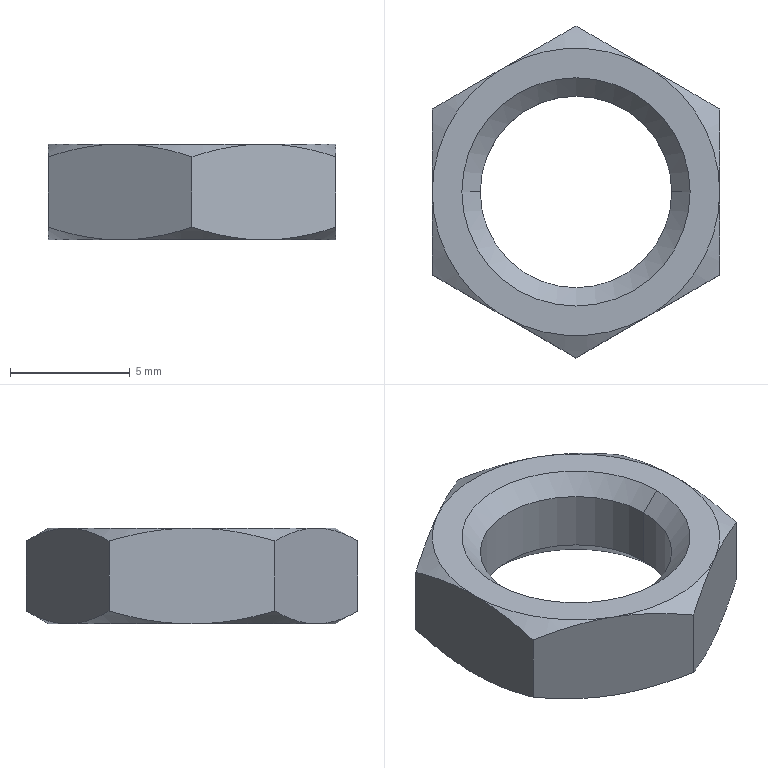Component | SolidWorks | RB0806-1_RB0806-3-1 | 1 solid | 26 faces | box 12 x 13.86 x 4 mm | volume 278 mm3 | cone 16 | plane 8 | cylinder 2 | commonest cylinder face diameters 8 x2
STEP:
#1=COLOUR_RGB('',0.7922,0.8196,0.9333);
#2=FILL_AREA_STYLE_COLOUR('',#1);
#3=FILL_AREA_STYLE('',(#2));
#4=SURFACE_STYLE_FILL_AREA(#3);
#5=SURFACE_SIDE_STYLE('',(#4));
#6=SURFACE_STYLE_USAGE(.BOTH.,#5);
#7=PRESENTATION_STYLE_ASSIGNMENT((#6));
#8=CARTESIAN_POINT('',(-0.6831,1.668,-1.143));
#9=VERTEX_POINT('',#8);
#10=CARTESIAN_POINT('',(-0.9981,1.668,-1.143));
#11=VERTEX_POINT('',#10);
#12=CARTESIAN_POINT('',(-0.8406,1.668,-1.143));
#13=DIRECTION('',(-0.,0.,1.));
#14=DIRECTION('',(-1.,0.,0.));
#15=AXIS2_PLACEMENT_3D('',#12,#13,#14);
#16=CIRCLE('',#15,0.1575);
#17=EDGE_CURVE('',#9,#11,#16,.T.);
#18=ORIENTED_EDGE('',*,*,#17,.F.);
#19=CARTESIAN_POINT('',(-0.653,1.668,-1.113));
#20=VERTEX_POINT('',#19);
#21=CARTESIAN_POINT('',(-0.668,1.668,-1.128));
#22=DIRECTION('',(0.7071,-0.,0.7071));
#23=VECTOR('',#22,39.37);
#24=LINE('',#21,#23);
#25=EDGE_CURVE('',#9,#20,#24,.T.);
#26=ORIENTED_EDGE('',*,*,#25,.T.);
#27=CARTESIAN_POINT('',(-1.028,1.668,-1.113));
#28=VERTEX_POINT('',#27);
#29=CARTESIAN_POINT('',(-0.8406,1.668,-1.113));
#30=DIRECTION('',(0.,-0.,-1.));
#31=DIRECTION('',(-1.,0.,0.));
#32=AXIS2_PLACEMENT_3D('',#29,#30,#31);
#33=CIRCLE('',#32,0.1876);
#34=EDGE_CURVE('',#28,#20,#33,.T.);
#35=ORIENTED_EDGE('',*,*,#34,.F.);
#36=CARTESIAN_POINT('',(-1.013,1.668,-1.128));
#37=DIRECTION('',(-0.7071,0.,0.7071));
#38=VECTOR('',#37,39.37);
#39=LINE('',#36,#38);
#40=EDGE_CURVE('',#11,#28,#39,.T.);
#41=ORIENTED_EDGE('',*,*,#40,.F.);
#42=EDGE_LOOP('',(#18,#26,#35,#41));
#43=FACE_OUTER_BOUND('',#42,.T.);
#44=CARTESIAN_POINT('',(-0.8406,1.668,-1.128));
#45=DIRECTION('',(-0.,0.,1.));
#46=DIRECTION('',(-1.,0.,0.));
#47=AXIS2_PLACEMENT_3D('',#44,#45,#46);
#48=CONICAL_SURFACE('',#47,0.1726,0.7854);
#49=ADVANCED_FACE('',(#43),#48,.F.);
#50=CARTESIAN_POINT('',(-0.6831,1.668,-1.24));
#51=VERTEX_POINT('',#50);
#52=CARTESIAN_POINT('',(-0.9981,1.668,-1.24));
#53=VERTEX_POINT('',#52);
#54=CARTESIAN_POINT('',(-0.8406,1.668,-1.24));
#55=DIRECTION('',(-0.,0.,1.));
#56=DIRECTION('',(1.,0.,0.));
#57=AXIS2_PLACEMENT_3D('',#54,#55,#56);
#58=CIRCLE('',#57,0.1575);
#59=EDGE_CURVE('',#51,#53,#58,.T.);
#60=ORIENTED_EDGE('',*,*,#59,.F.);
#61=CARTESIAN_POINT('',(-0.6831,1.668,-1.192));
#62=DIRECTION('',(-0.,0.,1.));
#63=VECTOR('',#62,39.37);
#64=LINE('',#61,#63);
#65=EDGE_CURVE('',#51,#9,#64,.T.);
#66=ORIENTED_EDGE('',*,*,#65,.T.);
#67=ORIENTED_EDGE('',*,*,#17,.T.);
#68=CARTESIAN_POINT('',(-0.9981,1.668,-1.192));
#69=DIRECTION('',(-0.,0.,1.));
#70=VECTOR('',#69,39.37);
#71=LINE('',#68,#70);
#72=EDGE_CURVE('',#53,#11,#71,.T.);
#73=ORIENTED_EDGE('',*,*,#72,.F.);
#74=EDGE_LOOP('',(#60,#66,#67,#73));
#75=FACE_OUTER_BOUND('',#74,.T.);
#76=CARTESIAN_POINT('',(-0.8406,1.668,-1.192));
#77=DIRECTION('',(-0.,0.,1.));
#78=DIRECTION('',(-1.,0.,0.));
#79=AXIS2_PLACEMENT_3D('',#76,#77,#78);
#80=CYLINDRICAL_SURFACE('',#79,0.1575);
#81=ADVANCED_FACE('',(#75),#80,.F.);
#82=ORIENTED_EDGE('',*,*,#59,.T.);
#83=CARTESIAN_POINT('',(-1.028,1.668,-1.27));
#84=VERTEX_POINT('',#83);
#85=CARTESIAN_POINT('',(-1.013,1.668,-1.255));
#86=DIRECTION('',(-0.7071,-0.,-0.7071));
#87=VECTOR('',#86,39.37);
#88=LINE('',#85,#87);
#89=EDGE_CURVE('',#53,#84,#88,.T.);
#90=ORIENTED_EDGE('',*,*,#89,.T.);
#91=CARTESIAN_POINT('',(-0.653,1.668,-1.27));
#92=VERTEX_POINT('',#91);
#93=CARTESIAN_POINT('',(-0.8406,1.668,-1.27));
#94=DIRECTION('',(-0.,0.,1.));
#95=DIRECTION('',(1.,0.,0.));
#96=AXIS2_PLACEMENT_3D('',#93,#94,#95);
#97=CIRCLE('',#96,0.1876);
#98=EDGE_CURVE('',#92,#84,#97,.T.);
#99=ORIENTED_EDGE('',*,*,#98,.F.);
#100=CARTESIAN_POINT('',(-0.668,1.668,-1.255));
#101=DIRECTION('',(0.7071,-0.,-0.7071));
#102=VECTOR('',#101,39.37);
#103=LINE('',#100,#102);
#104=EDGE_CURVE('',#51,#92,#103,.T.);
#105=ORIENTED_EDGE('',*,*,#104,.F.);
#106=EDGE_LOOP('',(#82,#90,#99,#105));
#107=FACE_OUTER_BOUND('',#106,.T.);
#108=CARTESIAN_POINT('',(-0.8406,1.668,-1.255));
#109=DIRECTION('',(0.,-0.,-1.));
#110=DIRECTION('',(1.,0.,0.));
#111=AXIS2_PLACEMENT_3D('',#108,#109,#110);
#112=CONICAL_SURFACE('',#111,0.1726,0.7854);
#113=ADVANCED_FACE('',(#107),#112,.F.);
#114=ORIENTED_EDGE('',*,*,#34,.T.);
#115=CARTESIAN_POINT('',(-0.8406,1.668,-1.113));
#116=DIRECTION('',(0.,-0.,-1.));
#117=DIRECTION('',(-1.,0.,0.));
#118=AXIS2_PLACEMENT_3D('',#115,#116,#117);
#119=CIRCLE('',#118,0.1876);
#120=EDGE_CURVE('',#20,#28,#119,.T.);
#121=ORIENTED_EDGE('',*,*,#120,.T.);
#122=EDGE_LOOP('',(#114,#121));
#123=FACE_BOUND('',#122,.T.);
#124=CARTESIAN_POINT('',(-0.6044,1.668,-1.113));
#125=VERTEX_POINT('',#124);
#126=CARTESIAN_POINT('',(-0.7225,1.872,-1.113));
#127=VERTEX_POINT('',#126);
#128=CARTESIAN_POINT('',(-0.8406,1.668,-1.113));
#129=DIRECTION('',(-0.,0.,1.));
#130=DIRECTION('',(1.,0.,0.));
#131=AXIS2_PLACEMENT_3D('',#128,#129,#130);
#132=CIRCLE('',#131,0.2362);
#133=EDGE_CURVE('',#125,#127,#132,.T.);
#134=ORIENTED_EDGE('',*,*,#133,.T.);
#135=CARTESIAN_POINT('',(-0.9587,1.872,-1.113));
#136=VERTEX_POINT('',#135);
#137=CARTESIAN_POINT('',(-0.8406,1.668,-1.113));
#138=DIRECTION('',(-0.,0.,1.));
#139=DIRECTION('',(1.,0.,0.));
#140=AXIS2_PLACEMENT_3D('',#137,#138,#139);
#141=CIRCLE('',#140,0.2362);
#142=EDGE_CURVE('',#127,#136,#141,.T.);
#143=ORIENTED_EDGE('',*,*,#142,.T.);
#144=CARTESIAN_POINT('',(-1.077,1.668,-1.113));
#145=VERTEX_POINT('',#144);
#146=CARTESIAN_POINT('',(-0.8406,1.668,-1.113));
#147=DIRECTION('',(-0.,0.,1.));
#148=DIRECTION('',(1.,0.,0.));
#149=AXIS2_PLACEMENT_3D('',#146,#147,#148);
#150=CIRCLE('',#149,0.2362);
#151=EDGE_CURVE('',#136,#145,#150,.T.);
#152=ORIENTED_EDGE('',*,*,#151,.T.);
#153=CARTESIAN_POINT('',(-0.9587,1.463,-1.113));
#154=VERTEX_POINT('',#153);
#155=CARTESIAN_POINT('',(-0.8406,1.668,-1.113));
#156=DIRECTION('',(-0.,0.,1.));
#157=DIRECTION('',(1.,0.,0.));
#158=AXIS2_PLACEMENT_3D('',#155,#156,#157);
#159=CIRCLE('',#158,0.2362);
#160=EDGE_CURVE('',#145,#154,#159,.T.);
#161=ORIENTED_EDGE('',*,*,#160,.T.);
#162=CARTESIAN_POINT('',(-0.7225,1.463,-1.113));
#163=VERTEX_POINT('',#162);
#164=CARTESIAN_POINT('',(-0.8406,1.668,-1.113));
#165=DIRECTION('',(-0.,0.,1.));
#166=DIRECTION('',(1.,-0.,0.));
#167=AXIS2_PLACEMENT_3D('',#164,#165,#166);
#168=CIRCLE('',#167,0.2362);
#169=EDGE_CURVE('',#154,#163,#168,.T.);
#170=ORIENTED_EDGE('',*,*,#169,.T.);
#171=CARTESIAN_POINT('',(-0.8406,1.668,-1.113));
#172=DIRECTION('',(-0.,0.,1.));
#173=DIRECTION('',(1.,-0.,0.));
#174=AXIS2_PLACEMENT_3D('',#171,#172,#173);
#175=CIRCLE('',#174,0.2362);
#176=EDGE_CURVE('',#163,#125,#175,.T.);
#177=ORIENTED_EDGE('',*,*,#176,.T.);
#178=EDGE_LOOP('',(#134,#143,#152,#161,#170,#177));
#179=FACE_OUTER_BOUND('',#178,.T.);
#180=CARTESIAN_POINT('',(-0.8406,1.865,-1.113));
#181=DIRECTION('',(-0.,0.,1.));
#182=DIRECTION('',(-1.,0.,-0.));
#183=AXIS2_PLACEMENT_3D('',#180,#181,#182);
#184=PLANE('',#183);
#185=ADVANCED_FACE('',(#123,#179),#184,.T.);
#186=ORIENTED_EDGE('',*,*,#25,.F.);
#187=CARTESIAN_POINT('',(-0.8406,1.668,-1.143));
#188=DIRECTION('',(-0.,0.,1.));
#189=DIRECTION('',(-1.,0.,0.));
#190=AXIS2_PLACEMENT_3D('',#187,#188,#189);
#191=CIRCLE('',#190,0.1575);
#192=EDGE_CURVE('',#11,#9,#191,.T.);
#193=ORIENTED_EDGE('',*,*,#192,.F.);
#194=ORIENTED_EDGE('',*,*,#40,.T.);
#195=ORIENTED_EDGE('',*,*,#120,.F.);
#196=EDGE_LOOP('',(#186,#193,#194,#195));
#197=FACE_OUTER_BOUND('',#196,.T.);
#198=CARTESIAN_POINT('',(-0.8406,1.668,-1.128));
#199=DIRECTION('',(-0.,0.,1.));
#200=DIRECTION('',(-1.,0.,0.));
#201=AXIS2_PLACEMENT_3D('',#198,#199,#200);
#202=CONICAL_SURFACE('',#201,0.1726,0.7854);
#203=ADVANCED_FACE('',(#197),#202,.F.);
#204=ORIENTED_EDGE('',*,*,#142,.F.);
#205=CARTESIAN_POINT('',(-0.8406,1.941,-1.134));
#206=VERTEX_POINT('',#205);
#207=CARTESIAN_POINT('',(-0.7225,1.872,-1.113));
#208=CARTESIAN_POINT('',(-0.7628,1.896,-1.113));
#209=CARTESIAN_POINT('',(-0.802,1.918,-1.121));
#210=CARTESIAN_POINT('',(-0.8406,1.941,-1.134));
#211=B_SPLINE_CURVE_WITH_KNOTS('',3,(#207,#208,#209,#210),.UNSPECIFIED.,.F.,.F.,(4,4),(0.,0.003505),.UNSPECIFIED.);
#212=EDGE_CURVE('',#127,#206,#211,.T.);
#213=ORIENTED_EDGE('',*,*,#212,.T.);
#214=CARTESIAN_POINT('',(-0.8406,1.941,-1.134));
#215=CARTESIAN_POINT('',(-0.8792,1.918,-1.121));
#216=CARTESIAN_POINT('',(-0.9184,1.896,-1.113));
#217=CARTESIAN_POINT('',(-0.9587,1.872,-1.113));
#218=B_SPLINE_CURVE_WITH_KNOTS('',3,(#214,#215,#216,#217),.UNSPECIFIED.,.F.,.F.,(4,4),(0.,0.003505),.UNSPECIFIED.);
#219=EDGE_CURVE('',#206,#136,#218,.T.);
#220=ORIENTED_EDGE('',*,*,#219,.T.);
#221=EDGE_LOOP('',(#204,#213,#220));
#222=FACE_OUTER_BOUND('',#221,.T.);
#223=CARTESIAN_POINT('',(-0.8406,1.668,-1.134));
#224=DIRECTION('',(0.,-0.,-1.));
#225=DIRECTION('',(1.,0.,0.));
#226=AXIS2_PLACEMENT_3D('',#223,#224,#225);
#227=CONICAL_SURFACE('',#226,0.273,1.047);
#228=ADVANCED_FACE('',(#222),#227,.T.);
#229=CARTESIAN_POINT('',(-0.6044,1.804,-1.134));
#230=VERTEX_POINT('',#229);
#231=CARTESIAN_POINT('',(-0.6044,1.804,-1.134));
#232=CARTESIAN_POINT('',(-0.6429,1.827,-1.121));
#233=CARTESIAN_POINT('',(-0.6822,1.849,-1.113));
#234=CARTESIAN_POINT('',(-0.7225,1.872,-1.113));
#235=B_SPLINE_CURVE_WITH_KNOTS('',3,(#231,#232,#233,#234),.UNSPECIFIED.,.F.,.F.,(4,4),(0.,0.003505),.UNSPECIFIED.);
#236=EDGE_CURVE('',#230,#127,#235,.T.);
#237=ORIENTED_EDGE('',*,*,#236,.T.);
#238=ORIENTED_EDGE('',*,*,#133,.F.);
#239=CARTESIAN_POINT('',(-0.6044,1.668,-1.113));
#240=CARTESIAN_POINT('',(-0.6044,1.714,-1.113));
#241=CARTESIAN_POINT('',(-0.6044,1.76,-1.121));
#242=CARTESIAN_POINT('',(-0.6044,1.804,-1.134));
#243=B_SPLINE_CURVE_WITH_KNOTS('',3,(#239,#240,#241,#242),.UNSPECIFIED.,.F.,.F.,(4,4),(0.,0.003505),.UNSPECIFIED.);
#244=EDGE_CURVE('',#125,#230,#243,.T.);
#245=ORIENTED_EDGE('',*,*,#244,.T.);
#246=EDGE_LOOP('',(#237,#238,#245));
#247=FACE_OUTER_BOUND('',#246,.T.);
#248=CARTESIAN_POINT('',(-0.8406,1.668,-1.134));
#249=DIRECTION('',(0.,-0.,-1.));
#250=DIRECTION('',(1.,0.,0.));
#251=AXIS2_PLACEMENT_3D('',#248,#249,#250);
#252=CONICAL_SURFACE('',#251,0.273,1.047);
#253=ADVANCED_FACE('',(#247),#252,.T.);
#254=ORIENTED_EDGE('',*,*,#176,.F.);
#255=CARTESIAN_POINT('',(-0.6044,1.532,-1.134));
#256=VERTEX_POINT('',#255);
#257=CARTESIAN_POINT('',(-0.7225,1.463,-1.113));
#258=CARTESIAN_POINT('',(-0.6822,1.487,-1.113));
#259=CARTESIAN_POINT('',(-0.6429,1.509,-1.121));
#260=CARTESIAN_POINT('',(-0.6044,1.532,-1.134));
#261=B_SPLINE_CURVE_WITH_KNOTS('',3,(#257,#258,#259,#260),.UNSPECIFIED.,.F.,.F.,(4,4),(0.,0.003505),.UNSPECIFIED.);
#262=EDGE_CURVE('',#163,#256,#261,.T.);
#263=ORIENTED_EDGE('',*,*,#262,.T.);
#264=CARTESIAN_POINT('',(-0.6044,1.532,-1.134));
#265=CARTESIAN_POINT('',(-0.6044,1.576,-1.121));
#266=CARTESIAN_POINT('',(-0.6044,1.621,-1.113));
#267=CARTESIAN_POINT('',(-0.6044,1.668,-1.113));
#268=B_SPLINE_CURVE_WITH_KNOTS('',3,(#264,#265,#266,#267),.UNSPECIFIED.,.F.,.F.,(4,4),(0.,0.003505),.UNSPECIFIED.);
#269=EDGE_CURVE('',#256,#125,#268,.T.);
#270=ORIENTED_EDGE('',*,*,#269,.T.);
#271=EDGE_LOOP('',(#254,#263,#270));
#272=FACE_OUTER_BOUND('',#271,.T.);
#273=CARTESIAN_POINT('',(-0.8406,1.668,-1.134));
#274=DIRECTION('',(0.,-0.,-1.));
#275=DIRECTION('',(1.,0.,0.));
#276=AXIS2_PLACEMENT_3D('',#273,#274,#275);
#277=CONICAL_SURFACE('',#276,0.273,1.047);
#278=ADVANCED_FACE('',(#272),#277,.T.);
#279=CARTESIAN_POINT('',(-0.8406,1.395,-1.134));
#280=VERTEX_POINT('',#279);
#281=CARTESIAN_POINT('',(-0.8406,1.395,-1.134));
#282=CARTESIAN_POINT('',(-0.802,1.417,-1.121));
#283=CARTESIAN_POINT('',(-0.7628,1.44,-1.113));
#284=CARTESIAN_POINT('',(-0.7225,1.463,-1.113));
#285=B_SPLINE_CURVE_WITH_KNOTS('',3,(#281,#282,#283,#284),.UNSPECIFIED.,.F.,.F.,(4,4),(0.,0.003505),.UNSPECIFIED.);
#286=EDGE_CURVE('',#280,#163,#285,.T.);
#287=ORIENTED_EDGE('',*,*,#286,.T.);
#288=ORIENTED_EDGE('',*,*,#169,.F.);
#289=CARTESIAN_POINT('',(-0.9587,1.463,-1.113));
#290=CARTESIAN_POINT('',(-0.9184,1.44,-1.113));
#291=CARTESIAN_POINT('',(-0.8792,1.417,-1.121));
#292=CARTESIAN_POINT('',(-0.8406,1.395,-1.134));
#293=B_SPLINE_CURVE_WITH_KNOTS('',3,(#289,#290,#291,#292),.UNSPECIFIED.,.F.,.F.,(4,4),(0.,0.003505),.UNSPECIFIED.);
#294=EDGE_CURVE('',#154,#280,#293,.T.);
#295=ORIENTED_EDGE('',*,*,#294,.T.);
#296=EDGE_LOOP('',(#287,#288,#295));
#297=FACE_OUTER_BOUND('',#296,.T.);
#298=CARTESIAN_POINT('',(-0.8406,1.668,-1.134));
#299=DIRECTION('',(0.,-0.,-1.));
#300=DIRECTION('',(1.,0.,0.));
#301=AXIS2_PLACEMENT_3D('',#298,#299,#300);
#302=CONICAL_SURFACE('',#301,0.273,1.047);
#303=ADVANCED_FACE('',(#297),#302,.T.);
#304=ORIENTED_EDGE('',*,*,#160,.F.);
#305=CARTESIAN_POINT('',(-1.077,1.532,-1.134));
#306=VERTEX_POINT('',#305);
#307=CARTESIAN_POINT('',(-1.077,1.668,-1.113));
#308=CARTESIAN_POINT('',(-1.077,1.621,-1.113));
#309=CARTESIAN_POINT('',(-1.077,1.576,-1.121));
#310=CARTESIAN_POINT('',(-1.077,1.532,-1.134));
#311=B_SPLINE_CURVE_WITH_KNOTS('',3,(#307,#308,#309,#310),.UNSPECIFIED.,.F.,.F.,(4,4),(0.,0.003505),.UNSPECIFIED.);
#312=EDGE_CURVE('',#145,#306,#311,.T.);
#313=ORIENTED_EDGE('',*,*,#312,.T.);
#314=CARTESIAN_POINT('',(-1.077,1.532,-1.134));
#315=CARTESIAN_POINT('',(-1.038,1.509,-1.121));
#316=CARTESIAN_POINT('',(-0.999,1.487,-1.113));
#317=CARTESIAN_POINT('',(-0.9587,1.463,-1.113));
#318=B_SPLINE_CURVE_WITH_KNOTS('',3,(#314,#315,#316,#317),.UNSPECIFIED.,.F.,.F.,(4,4),(0.,0.003505),.UNSPECIFIED.);
#319=EDGE_CURVE('',#306,#154,#318,.T.);
#320=ORIENTED_EDGE('',*,*,#319,.T.);
#321=EDGE_LOOP('',(#304,#313,#320));
#322=FACE_OUTER_BOUND('',#321,.T.);
#323=CARTESIAN_POINT('',(-0.8406,1.668,-1.134));
#324=DIRECTION('',(0.,-0.,-1.));
#325=DIRECTION('',(1.,0.,0.));
#326=AXIS2_PLACEMENT_3D('',#323,#324,#325);
#327=CONICAL_SURFACE('',#326,0.273,1.047);
#328=ADVANCED_FACE('',(#322),#327,.T.);
#329=CARTESIAN_POINT('',(-1.077,1.804,-1.134));
#330=VERTEX_POINT('',#329);
#331=CARTESIAN_POINT('',(-1.077,1.804,-1.134));
#332=CARTESIAN_POINT('',(-1.077,1.76,-1.121));
#333=CARTESIAN_POINT('',(-1.077,1.714,-1.113));
#334=CARTESIAN_POINT('',(-1.077,1.668,-1.113));
#335=B_SPLINE_CURVE_WITH_KNOTS('',3,(#331,#332,#333,#334),.UNSPECIFIED.,.F.,.F.,(4,4),(0.,0.003505),.UNSPECIFIED.);
#336=EDGE_CURVE('',#330,#145,#335,.T.);
#337=ORIENTED_EDGE('',*,*,#336,.T.);
#338=ORIENTED_EDGE('',*,*,#151,.F.);
#339=CARTESIAN_POINT('',(-0.9587,1.872,-1.113));
#340=CARTESIAN_POINT('',(-0.999,1.849,-1.113));
#341=CARTESIAN_POINT('',(-1.038,1.827,-1.121));
#342=CARTESIAN_POINT('',(-1.077,1.804,-1.134));
#343=B_SPLINE_CURVE_WITH_KNOTS('',3,(#339,#340,#341,#342),.UNSPECIFIED.,.F.,.F.,(4,4),(0.,0.003505),.UNSPECIFIED.);
#344=EDGE_CURVE('',#136,#330,#343,.T.);
#345=ORIENTED_EDGE('',*,*,#344,.T.);
#346=EDGE_LOOP('',(#337,#338,#345));
#347=FACE_OUTER_BOUND('',#346,.T.);
#348=CARTESIAN_POINT('',(-0.8406,1.668,-1.134));
#349=DIRECTION('',(0.,-0.,-1.));
#350=DIRECTION('',(1.,0.,0.));
#351=AXIS2_PLACEMENT_3D('',#348,#349,#350);
#352=CONICAL_SURFACE('',#351,0.273,1.047);
#353=ADVANCED_FACE('',(#347),#352,.T.);
#354=ORIENTED_EDGE('',*,*,#65,.F.);
#355=CARTESIAN_POINT('',(-0.8406,1.668,-1.24));
#356=DIRECTION('',(-0.,0.,1.));
#357=DIRECTION('',(1.,0.,0.));
#358=AXIS2_PLACEMENT_3D('',#355,#356,#357);
#359=CIRCLE('',#358,0.1575);
#360=EDGE_CURVE('',#53,#51,#359,.T.);
#361=ORIENTED_EDGE('',*,*,#360,.F.);
#362=ORIENTED_EDGE('',*,*,#72,.T.);
#363=ORIENTED_EDGE('',*,*,#192,.T.);
#364=EDGE_LOOP('',(#354,#361,#362,#363));
#365=FACE_OUTER_BOUND('',#364,.T.);
#366=CARTESIAN_POINT('',(-0.8406,1.668,-1.192));
#367=DIRECTION('',(-0.,0.,1.));
#368=DIRECTION('',(-1.,0.,0.));
#369=AXIS2_PLACEMENT_3D('',#366,#367,#368);
#370=CYLINDRICAL_SURFACE('',#369,0.1575);
#371=ADVANCED_FACE('',(#365),#370,.F.);
#372=CARTESIAN_POINT('',(-0.6044,1.804,-1.249));
#373=VERTEX_POINT('',#372);
#374=CARTESIAN_POINT('',(-0.6044,1.804,-1.27));
#375=DIRECTION('',(-0.,0.,1.));
#376=VECTOR('',#375,39.37);
#377=LINE('',#374,#376);
#378=EDGE_CURVE('',#373,#230,#377,.T.);
#379=ORIENTED_EDGE('',*,*,#378,.F.);
#380=CARTESIAN_POINT('',(-0.7225,1.872,-1.27));
#381=VERTEX_POINT('',#380);
#382=CARTESIAN_POINT('',(-0.7225,1.872,-1.27));
#383=CARTESIAN_POINT('',(-0.6822,1.849,-1.27));
#384=CARTESIAN_POINT('',(-0.6429,1.827,-1.262));
#385=CARTESIAN_POINT('',(-0.6044,1.804,-1.249));
#386=B_SPLINE_CURVE_WITH_KNOTS('',3,(#382,#383,#384,#385),.UNSPECIFIED.,.F.,.F.,(4,4),(0.,0.003505),.UNSPECIFIED.);
#387=EDGE_CURVE('',#381,#373,#386,.T.);
#388=ORIENTED_EDGE('',*,*,#387,.F.);
#389=CARTESIAN_POINT('',(-0.8406,1.941,-1.249));
#390=VERTEX_POINT('',#389);
#391=CARTESIAN_POINT('',(-0.8406,1.941,-1.249));
#392=CARTESIAN_POINT('',(-0.802,1.918,-1.262));
#393=CARTESIAN_POINT('',(-0.7628,1.896,-1.27));
#394=CARTESIAN_POINT('',(-0.7225,1.872,-1.27));
#395=B_SPLINE_CURVE_WITH_KNOTS('',3,(#391,#392,#393,#394),.UNSPECIFIED.,.F.,.F.,(4,4),(0.,0.003505),.UNSPECIFIED.);
#396=EDGE_CURVE('',#390,#381,#395,.T.);
#397=ORIENTED_EDGE('',*,*,#396,.F.);
#398=CARTESIAN_POINT('',(-0.8406,1.941,-1.27));
#399=DIRECTION('',(0.,-0.,-1.));
#400=VECTOR('',#399,39.37);
#401=LINE('',#398,#400);
#402=EDGE_CURVE('',#206,#390,#401,.T.);
#403=ORIENTED_EDGE('',*,*,#402,.F.);
#404=ORIENTED_EDGE('',*,*,#212,.F.);
#405=ORIENTED_EDGE('',*,*,#236,.F.);
#406=EDGE_LOOP('',(#379,#388,#397,#403,#404,#405));
#407=FACE_OUTER_BOUND('',#406,.T.);
#408=CARTESIAN_POINT('',(-0.6044,1.804,-1.27));
#409=DIRECTION('',(-0.5,-0.866,0.));
#410=DIRECTION('',(-0.866,0.5,-0.));
#411=AXIS2_PLACEMENT_3D('',#408,#409,#410);
#412=PLANE('',#411);
#413=ADVANCED_FACE('',(#407),#412,.F.);
#414=CARTESIAN_POINT('',(-0.6044,1.532,-1.249));
#415=VERTEX_POINT('',#414);
#416=CARTESIAN_POINT('',(-0.6044,1.532,-1.27));
#417=DIRECTION('',(-0.,0.,1.));
#418=VECTOR('',#417,39.37);
#419=LINE('',#416,#418);
#420=EDGE_CURVE('',#415,#256,#419,.T.);
#421=ORIENTED_EDGE('',*,*,#420,.F.);
#422=CARTESIAN_POINT('',(-0.6044,1.668,-1.27));
#423=VERTEX_POINT('',#422);
#424=CARTESIAN_POINT('',(-0.6044,1.668,-1.27));
#425=CARTESIAN_POINT('',(-0.6044,1.621,-1.27));
#426=CARTESIAN_POINT('',(-0.6044,1.576,-1.262));
#427=CARTESIAN_POINT('',(-0.6044,1.532,-1.249));
#428=B_SPLINE_CURVE_WITH_KNOTS('',3,(#424,#425,#426,#427),.UNSPECIFIED.,.F.,.F.,(4,4),(0.,0.003505),.UNSPECIFIED.);
#429=EDGE_CURVE('',#423,#415,#428,.T.);
#430=ORIENTED_EDGE('',*,*,#429,.F.);
#431=CARTESIAN_POINT('',(-0.6044,1.804,-1.249));
#432=CARTESIAN_POINT('',(-0.6044,1.76,-1.262));
#433=CARTESIAN_POINT('',(-0.6044,1.714,-1.27));
#434=CARTESIAN_POINT('',(-0.6044,1.668,-1.27));
#435=B_SPLINE_CURVE_WITH_KNOTS('',3,(#431,#432,#433,#434),.UNSPECIFIED.,.F.,.F.,(4,4),(0.,0.003505),.UNSPECIFIED.);
#436=EDGE_CURVE('',#373,#423,#435,.T.);
#437=ORIENTED_EDGE('',*,*,#436,.F.);
#438=ORIENTED_EDGE('',*,*,#378,.T.);
#439=ORIENTED_EDGE('',*,*,#244,.F.);
#440=ORIENTED_EDGE('',*,*,#269,.F.);
#441=EDGE_LOOP('',(#421,#430,#437,#438,#439,#440));
#442=FACE_OUTER_BOUND('',#441,.T.);
#443=CARTESIAN_POINT('',(-0.6044,1.532,-1.27));
#444=DIRECTION('',(-1.,0.,-0.));
#445=DIRECTION('',(0.,-0.,-1.));
#446=AXIS2_PLACEMENT_3D('',#443,#444,#445);
#447=PLANE('',#446);
#448=ADVANCED_FACE('',(#442),#447,.F.);
#449=ORIENTED_EDGE('',*,*,#286,.F.);
#450=CARTESIAN_POINT('',(-0.8406,1.395,-1.249));
#451=VERTEX_POINT('',#450);
#452=CARTESIAN_POINT('',(-0.8406,1.395,-1.27));
#453=DIRECTION('',(-0.,0.,1.));
#454=VECTOR('',#453,39.37);
#455=LINE('',#452,#454);
#456=EDGE_CURVE('',#451,#280,#455,.T.);
#457=ORIENTED_EDGE('',*,*,#456,.F.);
#458=CARTESIAN_POINT('',(-0.7225,1.463,-1.27));
#459=VERTEX_POINT('',#458);
#460=CARTESIAN_POINT('',(-0.7225,1.463,-1.27));
#461=CARTESIAN_POINT('',(-0.7628,1.44,-1.27));
#462=CARTESIAN_POINT('',(-0.802,1.417,-1.262));
#463=CARTESIAN_POINT('',(-0.8406,1.395,-1.249));
#464=B_SPLINE_CURVE_WITH_KNOTS('',3,(#460,#461,#462,#463),.UNSPECIFIED.,.F.,.F.,(4,4),(0.,0.003505),.UNSPECIFIED.);
#465=EDGE_CURVE('',#459,#451,#464,.T.);
#466=ORIENTED_EDGE('',*,*,#465,.F.);
#467=CARTESIAN_POINT('',(-0.6044,1.532,-1.249));
#468=CARTESIAN_POINT('',(-0.6429,1.509,-1.262));
#469=CARTESIAN_POINT('',(-0.6822,1.487,-1.27));
#470=CARTESIAN_POINT('',(-0.7225,1.463,-1.27));
#471=B_SPLINE_CURVE_WITH_KNOTS('',3,(#467,#468,#469,#470),.UNSPECIFIED.,.F.,.F.,(4,4),(0.,0.003505),.UNSPECIFIED.);
#472=EDGE_CURVE('',#415,#459,#471,.T.);
#473=ORIENTED_EDGE('',*,*,#472,.F.);
#474=ORIENTED_EDGE('',*,*,#420,.T.);
#475=ORIENTED_EDGE('',*,*,#262,.F.);
#476=EDGE_LOOP('',(#449,#457,#466,#473,#474,#475));
#477=FACE_OUTER_BOUND('',#476,.T.);
#478=CARTESIAN_POINT('',(-0.8406,1.395,-1.27));
#479=DIRECTION('',(-0.5,0.866,-0.));
#480=DIRECTION('',(0.866,0.5,-0.));
#481=AXIS2_PLACEMENT_3D('',#478,#479,#480);
#482=PLANE('',#481);
#483=ADVANCED_FACE('',(#477),#482,.F.);
#484=ORIENTED_EDGE('',*,*,#319,.F.);
#485=CARTESIAN_POINT('',(-1.077,1.532,-1.249));
#486=VERTEX_POINT('',#485);
#487=CARTESIAN_POINT('',(-1.077,1.532,-1.27));
#488=DIRECTION('',(-0.,0.,1.));
#489=VECTOR('',#488,39.37);
#490=LINE('',#487,#489);
#491=EDGE_CURVE('',#486,#306,#490,.T.);
#492=ORIENTED_EDGE('',*,*,#491,.F.);
#493=CARTESIAN_POINT('',(-0.9587,1.463,-1.27));
#494=VERTEX_POINT('',#493);
#495=CARTESIAN_POINT('',(-0.9587,1.463,-1.27));
#496=CARTESIAN_POINT('',(-0.999,1.487,-1.27));
#497=CARTESIAN_POINT('',(-1.038,1.509,-1.262));
#498=CARTESIAN_POINT('',(-1.077,1.532,-1.249));
#499=B_SPLINE_CURVE_WITH_KNOTS('',3,(#495,#496,#497,#498),.UNSPECIFIED.,.F.,.F.,(4,4),(0.,0.003505),.UNSPECIFIED.);
#500=EDGE_CURVE('',#494,#486,#499,.T.);
#501=ORIENTED_EDGE('',*,*,#500,.F.);
#502=CARTESIAN_POINT('',(-0.8406,1.395,-1.249));
#503=CARTESIAN_POINT('',(-0.8792,1.417,-1.262));
#504=CARTESIAN_POINT('',(-0.9184,1.44,-1.27));
#505=CARTESIAN_POINT('',(-0.9587,1.463,-1.27));
#506=B_SPLINE_CURVE_WITH_KNOTS('',3,(#502,#503,#504,#505),.UNSPECIFIED.,.F.,.F.,(4,4),(0.,0.003505),.UNSPECIFIED.);
#507=EDGE_CURVE('',#451,#494,#506,.T.);
#508=ORIENTED_EDGE('',*,*,#507,.F.);
#509=ORIENTED_EDGE('',*,*,#456,.T.);
#510=ORIENTED_EDGE('',*,*,#294,.F.);
#511=EDGE_LOOP('',(#484,#492,#501,#508,#509,#510));
#512=FACE_OUTER_BOUND('',#511,.T.);
#513=CARTESIAN_POINT('',(-1.077,1.532,-1.27));
#514=DIRECTION('',(0.5,0.866,-0.));
#515=DIRECTION('',(0.866,-0.5,0.));
#516=AXIS2_PLACEMENT_3D('',#513,#514,#515);
#517=PLANE('',#516);
#518=ADVANCED_FACE('',(#512),#517,.F.);
#519=ORIENTED_EDGE('',*,*,#336,.F.);
#520=CARTESIAN_POINT('',(-1.077,1.804,-1.249));
#521=VERTEX_POINT('',#520);
#522=CARTESIAN_POINT('',(-1.077,1.804,-1.27));
#523=DIRECTION('',(-0.,0.,1.));
#524=VECTOR('',#523,39.37);
#525=LINE('',#522,#524);
#526=EDGE_CURVE('',#521,#330,#525,.T.);
#527=ORIENTED_EDGE('',*,*,#526,.F.);
#528=CARTESIAN_POINT('',(-1.077,1.668,-1.27));
#529=VERTEX_POINT('',#528);
#530=CARTESIAN_POINT('',(-1.077,1.668,-1.27));
#531=CARTESIAN_POINT('',(-1.077,1.714,-1.27));
#532=CARTESIAN_POINT('',(-1.077,1.76,-1.262));
#533=CARTESIAN_POINT('',(-1.077,1.804,-1.249));
#534=B_SPLINE_CURVE_WITH_KNOTS('',3,(#530,#531,#532,#533),.UNSPECIFIED.,.F.,.F.,(4,4),(0.,0.003505),.UNSPECIFIED.);
#535=EDGE_CURVE('',#529,#521,#534,.T.);
#536=ORIENTED_EDGE('',*,*,#535,.F.);
#537=CARTESIAN_POINT('',(-1.077,1.532,-1.249));
#538=CARTESIAN_POINT('',(-1.077,1.576,-1.262));
#539=CARTESIAN_POINT('',(-1.077,1.621,-1.27));
#540=CARTESIAN_POINT('',(-1.077,1.668,-1.27));
#541=B_SPLINE_CURVE_WITH_KNOTS('',3,(#537,#538,#539,#540),.UNSPECIFIED.,.F.,.F.,(4,4),(0.,0.003505),.UNSPECIFIED.);
#542=EDGE_CURVE('',#486,#529,#541,.T.);
#543=ORIENTED_EDGE('',*,*,#542,.F.);
#544=ORIENTED_EDGE('',*,*,#491,.T.);
#545=ORIENTED_EDGE('',*,*,#312,.F.);
#546=EDGE_LOOP('',(#519,#527,#536,#543,#544,#545));
#547=FACE_OUTER_BOUND('',#546,.T.);
#548=CARTESIAN_POINT('',(-1.077,1.804,-1.27));
#549=DIRECTION('',(1.,-0.,0.));
#550=DIRECTION('',(-0.,0.,1.));
#551=AXIS2_PLACEMENT_3D('',#548,#549,#550);
#552=PLANE('',#551);
#553=ADVANCED_FACE('',(#547),#552,.F.);
#554=ORIENTED_EDGE('',*,*,#402,.T.);
#555=CARTESIAN_POINT('',(-0.9587,1.872,-1.27));
#556=VERTEX_POINT('',#555);
#557=CARTESIAN_POINT('',(-0.9587,1.872,-1.27));
#558=CARTESIAN_POINT('',(-0.9184,1.896,-1.27));
#559=CARTESIAN_POINT('',(-0.8792,1.918,-1.262));
#560=CARTESIAN_POINT('',(-0.8406,1.941,-1.249));
#561=B_SPLINE_CURVE_WITH_KNOTS('',3,(#557,#558,#559,#560),.UNSPECIFIED.,.F.,.F.,(4,4),(0.,0.003505),.UNSPECIFIED.);
#562=EDGE_CURVE('',#556,#390,#561,.T.);
#563=ORIENTED_EDGE('',*,*,#562,.F.);
#564=CARTESIAN_POINT('',(-1.077,1.804,-1.249));
#565=CARTESIAN_POINT('',(-1.038,1.827,-1.262));
#566=CARTESIAN_POINT('',(-0.999,1.849,-1.27));
#567=CARTESIAN_POINT('',(-0.9587,1.872,-1.27));
#568=B_SPLINE_CURVE_WITH_KNOTS('',3,(#564,#565,#566,#567),.UNSPECIFIED.,.F.,.F.,(4,4),(0.,0.003505),.UNSPECIFIED.);
#569=EDGE_CURVE('',#521,#556,#568,.T.);
#570=ORIENTED_EDGE('',*,*,#569,.F.);
#571=ORIENTED_EDGE('',*,*,#526,.T.);
#572=ORIENTED_EDGE('',*,*,#344,.F.);
#573=ORIENTED_EDGE('',*,*,#219,.F.);
#574=EDGE_LOOP('',(#554,#563,#570,#571,#572,#573));
#575=FACE_OUTER_BOUND('',#574,.T.);
#576=CARTESIAN_POINT('',(-0.8406,1.941,-1.27));
#577=DIRECTION('',(0.5,-0.866,0.));
#578=DIRECTION('',(-0.866,-0.5,0.));
#579=AXIS2_PLACEMENT_3D('',#576,#577,#578);
#580=PLANE('',#579);
#581=ADVANCED_FACE('',(#575),#580,.F.);
#582=ORIENTED_EDGE('',*,*,#89,.F.);
#583=ORIENTED_EDGE('',*,*,#360,.T.);
#584=ORIENTED_EDGE('',*,*,#104,.T.);
#585=CARTESIAN_POINT('',(-0.8406,1.668,-1.27));
#586=DIRECTION('',(-0.,0.,1.));
#587=DIRECTION('',(1.,0.,0.));
#588=AXIS2_PLACEMENT_3D('',#585,#586,#587);
#589=CIRCLE('',#588,0.1876);
#590=EDGE_CURVE('',#84,#92,#589,.T.);
#591=ORIENTED_EDGE('',*,*,#590,.F.);
#592=EDGE_LOOP('',(#582,#583,#584,#591));
#593=FACE_OUTER_BOUND('',#592,.T.);
#594=CARTESIAN_POINT('',(-0.8406,1.668,-1.255));
#595=DIRECTION('',(0.,-0.,-1.));
#596=DIRECTION('',(1.,0.,0.));
#597=AXIS2_PLACEMENT_3D('',#594,#595,#596);
#598=CONICAL_SURFACE('',#597,0.1726,0.7854);
#599=ADVANCED_FACE('',(#593),#598,.F.);
#600=CARTESIAN_POINT('',(-0.8406,1.668,-1.27));
#601=DIRECTION('',(0.,0.,1.));
#602=DIRECTION('',(-1.,0.,0.));
#603=AXIS2_PLACEMENT_3D('',#600,#601,#602);
#604=CIRCLE('',#603,0.2362);
#605=EDGE_CURVE('',#423,#381,#604,.T.);
#606=ORIENTED_EDGE('',*,*,#605,.T.);
#607=ORIENTED_EDGE('',*,*,#387,.T.);
#608=ORIENTED_EDGE('',*,*,#436,.T.);
#609=EDGE_LOOP('',(#606,#607,#608));
#610=FACE_OUTER_BOUND('',#609,.T.);
#611=CARTESIAN_POINT('',(-0.8406,1.668,-1.249));
#612=DIRECTION('',(0.,0.,1.));
#613=DIRECTION('',(-1.,0.,0.));
#614=AXIS2_PLACEMENT_3D('',#611,#612,#613);
#615=CONICAL_SURFACE('',#614,0.273,1.047);
#616=ADVANCED_FACE('',(#610),#615,.T.);
#617=ORIENTED_EDGE('',*,*,#396,.T.);
#618=CARTESIAN_POINT('',(-0.8406,1.668,-1.27));
#619=DIRECTION('',(-0.,0.,1.));
#620=DIRECTION('',(-1.,0.,0.));
#621=AXIS2_PLACEMENT_3D('',#618,#619,#620);
#622=CIRCLE('',#621,0.2362);
#623=EDGE_CURVE('',#381,#556,#622,.T.);
#624=ORIENTED_EDGE('',*,*,#623,.T.);
#625=ORIENTED_EDGE('',*,*,#562,.T.);
#626=EDGE_LOOP('',(#617,#624,#625));
#627=FACE_OUTER_BOUND('',#626,.T.);
#628=CARTESIAN_POINT('',(-0.8406,1.668,-1.249));
#629=DIRECTION('',(-0.,0.,1.));
#630=DIRECTION('',(-1.,0.,0.));
#631=AXIS2_PLACEMENT_3D('',#628,#629,#630);
#632=CONICAL_SURFACE('',#631,0.273,1.047);
#633=ADVANCED_FACE('',(#627),#632,.T.);
#634=CARTESIAN_POINT('',(-0.8406,1.668,-1.27));
#635=DIRECTION('',(0.,0.,1.));
#636=DIRECTION('',(-1.,0.,0.));
#637=AXIS2_PLACEMENT_3D('',#634,#635,#636);
#638=CIRCLE('',#637,0.2362);
#639=EDGE_CURVE('',#459,#423,#638,.T.);
#640=ORIENTED_EDGE('',*,*,#639,.T.);
#641=ORIENTED_EDGE('',*,*,#429,.T.);
#642=ORIENTED_EDGE('',*,*,#472,.T.);
#643=EDGE_LOOP('',(#640,#641,#642));
#644=FACE_OUTER_BOUND('',#643,.T.);
#645=CARTESIAN_POINT('',(-0.8406,1.668,-1.249));
#646=DIRECTION('',(0.,0.,1.));
#647=DIRECTION('',(-1.,0.,0.));
#648=AXIS2_PLACEMENT_3D('',#645,#646,#647);
#649=CONICAL_SURFACE('',#648,0.273,1.047);
#650=ADVANCED_FACE('',(#644),#649,.T.);
#651=CARTESIAN_POINT('',(-0.8406,1.668,-1.27));
#652=DIRECTION('',(-0.,0.,1.));
#653=DIRECTION('',(-1.,0.,0.));
#654=AXIS2_PLACEMENT_3D('',#651,#652,#653);
#655=CIRCLE('',#654,0.2362);
#656=EDGE_CURVE('',#494,#459,#655,.T.);
#657=ORIENTED_EDGE('',*,*,#656,.T.);
#658=ORIENTED_EDGE('',*,*,#465,.T.);
#659=ORIENTED_EDGE('',*,*,#507,.T.);
#660=EDGE_LOOP('',(#657,#658,#659));
#661=FACE_OUTER_BOUND('',#660,.T.);
#662=CARTESIAN_POINT('',(-0.8406,1.668,-1.249));
#663=DIRECTION('',(-0.,0.,1.));
#664=DIRECTION('',(-1.,0.,0.));
#665=AXIS2_PLACEMENT_3D('',#662,#663,#664);
#666=CONICAL_SURFACE('',#665,0.273,1.047);
#667=ADVANCED_FACE('',(#661),#666,.T.);
#668=ORIENTED_EDGE('',*,*,#542,.T.);
#669=CARTESIAN_POINT('',(-0.8406,1.668,-1.27));
#670=DIRECTION('',(0.,0.,1.));
#671=DIRECTION('',(-1.,0.,0.));
#672=AXIS2_PLACEMENT_3D('',#669,#670,#671);
#673=CIRCLE('',#672,0.2362);
#674=EDGE_CURVE('',#529,#494,#673,.T.);
#675=ORIENTED_EDGE('',*,*,#674,.T.);
#676=ORIENTED_EDGE('',*,*,#500,.T.);
#677=EDGE_LOOP('',(#668,#675,#676));
#678=FACE_OUTER_BOUND('',#677,.T.);
#679=CARTESIAN_POINT('',(-0.8406,1.668,-1.249));
#680=DIRECTION('',(0.,0.,1.));
#681=DIRECTION('',(-1.,0.,0.));
#682=AXIS2_PLACEMENT_3D('',#679,#680,#681);
#683=CONICAL_SURFACE('',#682,0.273,1.047);
#684=ADVANCED_FACE('',(#678),#683,.T.);
#685=ORIENTED_EDGE('',*,*,#569,.T.);
#686=CARTESIAN_POINT('',(-0.8406,1.668,-1.27));
#687=DIRECTION('',(0.,0.,1.));
#688=DIRECTION('',(-1.,0.,0.));
#689=AXIS2_PLACEMENT_3D('',#686,#687,#688);
#690=CIRCLE('',#689,0.2362);
#691=EDGE_CURVE('',#556,#529,#690,.T.);
#692=ORIENTED_EDGE('',*,*,#691,.T.);
#693=ORIENTED_EDGE('',*,*,#535,.T.);
#694=EDGE_LOOP('',(#685,#692,#693));
#695=FACE_OUTER_BOUND('',#694,.T.);
#696=CARTESIAN_POINT('',(-0.8406,1.668,-1.249));
#697=DIRECTION('',(0.,0.,1.));
#698=DIRECTION('',(-1.,0.,0.));
#699=AXIS2_PLACEMENT_3D('',#696,#697,#698);
#700=CONICAL_SURFACE('',#699,0.273,1.047);
#701=ADVANCED_FACE('',(#695),#700,.T.);
#702=ORIENTED_EDGE('',*,*,#674,.F.);
#703=ORIENTED_EDGE('',*,*,#691,.F.);
#704=ORIENTED_EDGE('',*,*,#623,.F.);
#705=ORIENTED_EDGE('',*,*,#605,.F.);
#706=ORIENTED_EDGE('',*,*,#639,.F.);
#707=ORIENTED_EDGE('',*,*,#656,.F.);
#708=EDGE_LOOP('',(#702,#703,#704,#705,#706,#707));
#709=FACE_OUTER_BOUND('',#708,.T.);
#710=ORIENTED_EDGE('',*,*,#98,.T.);
#711=ORIENTED_EDGE('',*,*,#590,.T.);
#712=EDGE_LOOP('',(#710,#711));
#713=FACE_BOUND('',#712,.T.);
#714=CARTESIAN_POINT('',(-0.8406,1.865,-1.27));
#715=DIRECTION('',(0.,-0.,-1.));
#716=DIRECTION('',(1.,-0.,0.));
#717=AXIS2_PLACEMENT_3D('',#714,#715,#716);
#718=PLANE('',#717);
#719=ADVANCED_FACE('',(#709,#713),#718,.T.);
#720=CLOSED_SHELL('',(#49,#81,#113,#185,#203,#228,#253,#278,#303,#328,#353,#371,#413,#448,#483,#518,#553,#581,#599,#616,#633,#650,#667,#684,#701,#719));
#721=MANIFOLD_SOLID_BREP('',#720);
#722=STYLED_ITEM('',(#7),#721);
#723=(LENGTH_UNIT()NAMED_UNIT(*)SI_UNIT($,.METRE.));
#724=LENGTH_MEASURE_WITH_UNIT(LENGTH_MEASURE(0.0254),#723);
#725=DIMENSIONAL_EXPONENTS(1.,0.,0.,0.,0.,0.,0.);
#726=(CONVERSION_BASED_UNIT('',#724)LENGTH_UNIT()NAMED_UNIT(#725));
#727=UNCERTAINTY_MEASURE_WITH_UNIT(LENGTH_MEASURE(0.00001),#726,'','');
#728=(NAMED_UNIT(*)PLANE_ANGLE_UNIT()SI_UNIT($,.RADIAN.));
#729=(NAMED_UNIT(*)SI_UNIT($,.STERADIAN.)SOLID_ANGLE_UNIT());
#730=(GEOMETRIC_REPRESENTATION_CONTEXT(3)GLOBAL_UNCERTAINTY_ASSIGNED_CONTEXT((#727))GLOBAL_UNIT_ASSIGNED_CONTEXT((#726,#728,#729))REPRESENTATION_CONTEXT('',''));
#731=MECHANICAL_DESIGN_GEOMETRIC_PRESENTATION_REPRESENTATION('',(#722),#730);
#732=CARTESIAN_POINT('',(0.,0.,0.));
#733=DIRECTION('',(0.,0.,1.));
#734=DIRECTION('',(1.,0.,0.));
#735=AXIS2_PLACEMENT_3D('',#732,#733,#734);
#736=(LENGTH_UNIT()NAMED_UNIT(*)SI_UNIT($,.METRE.));
#737=LENGTH_MEASURE_WITH_UNIT(LENGTH_MEASURE(0.0254),#736);
#738=DIMENSIONAL_EXPONENTS(1.,0.,0.,0.,0.,0.,0.);
#739=(CONVERSION_BASED_UNIT('',#737)LENGTH_UNIT()NAMED_UNIT(#738));
#740=UNCERTAINTY_MEASURE_WITH_UNIT(LENGTH_MEASURE(0.00001),#739,'','');
#741=(NAMED_UNIT(*)PLANE_ANGLE_UNIT()SI_UNIT($,.RADIAN.));
#742=(NAMED_UNIT(*)SI_UNIT($,.STERADIAN.)SOLID_ANGLE_UNIT());
#743=(GEOMETRIC_REPRESENTATION_CONTEXT(3)GLOBAL_UNCERTAINTY_ASSIGNED_CONTEXT((#740))GLOBAL_UNIT_ASSIGNED_CONTEXT((#739,#741,#742))REPRESENTATION_CONTEXT('',''));
#744=ADVANCED_BREP_SHAPE_REPRESENTATION('',(#721,#735),#743);
#745=PRESENTATION_LAYER_ASSIGNMENT('','',(#722));